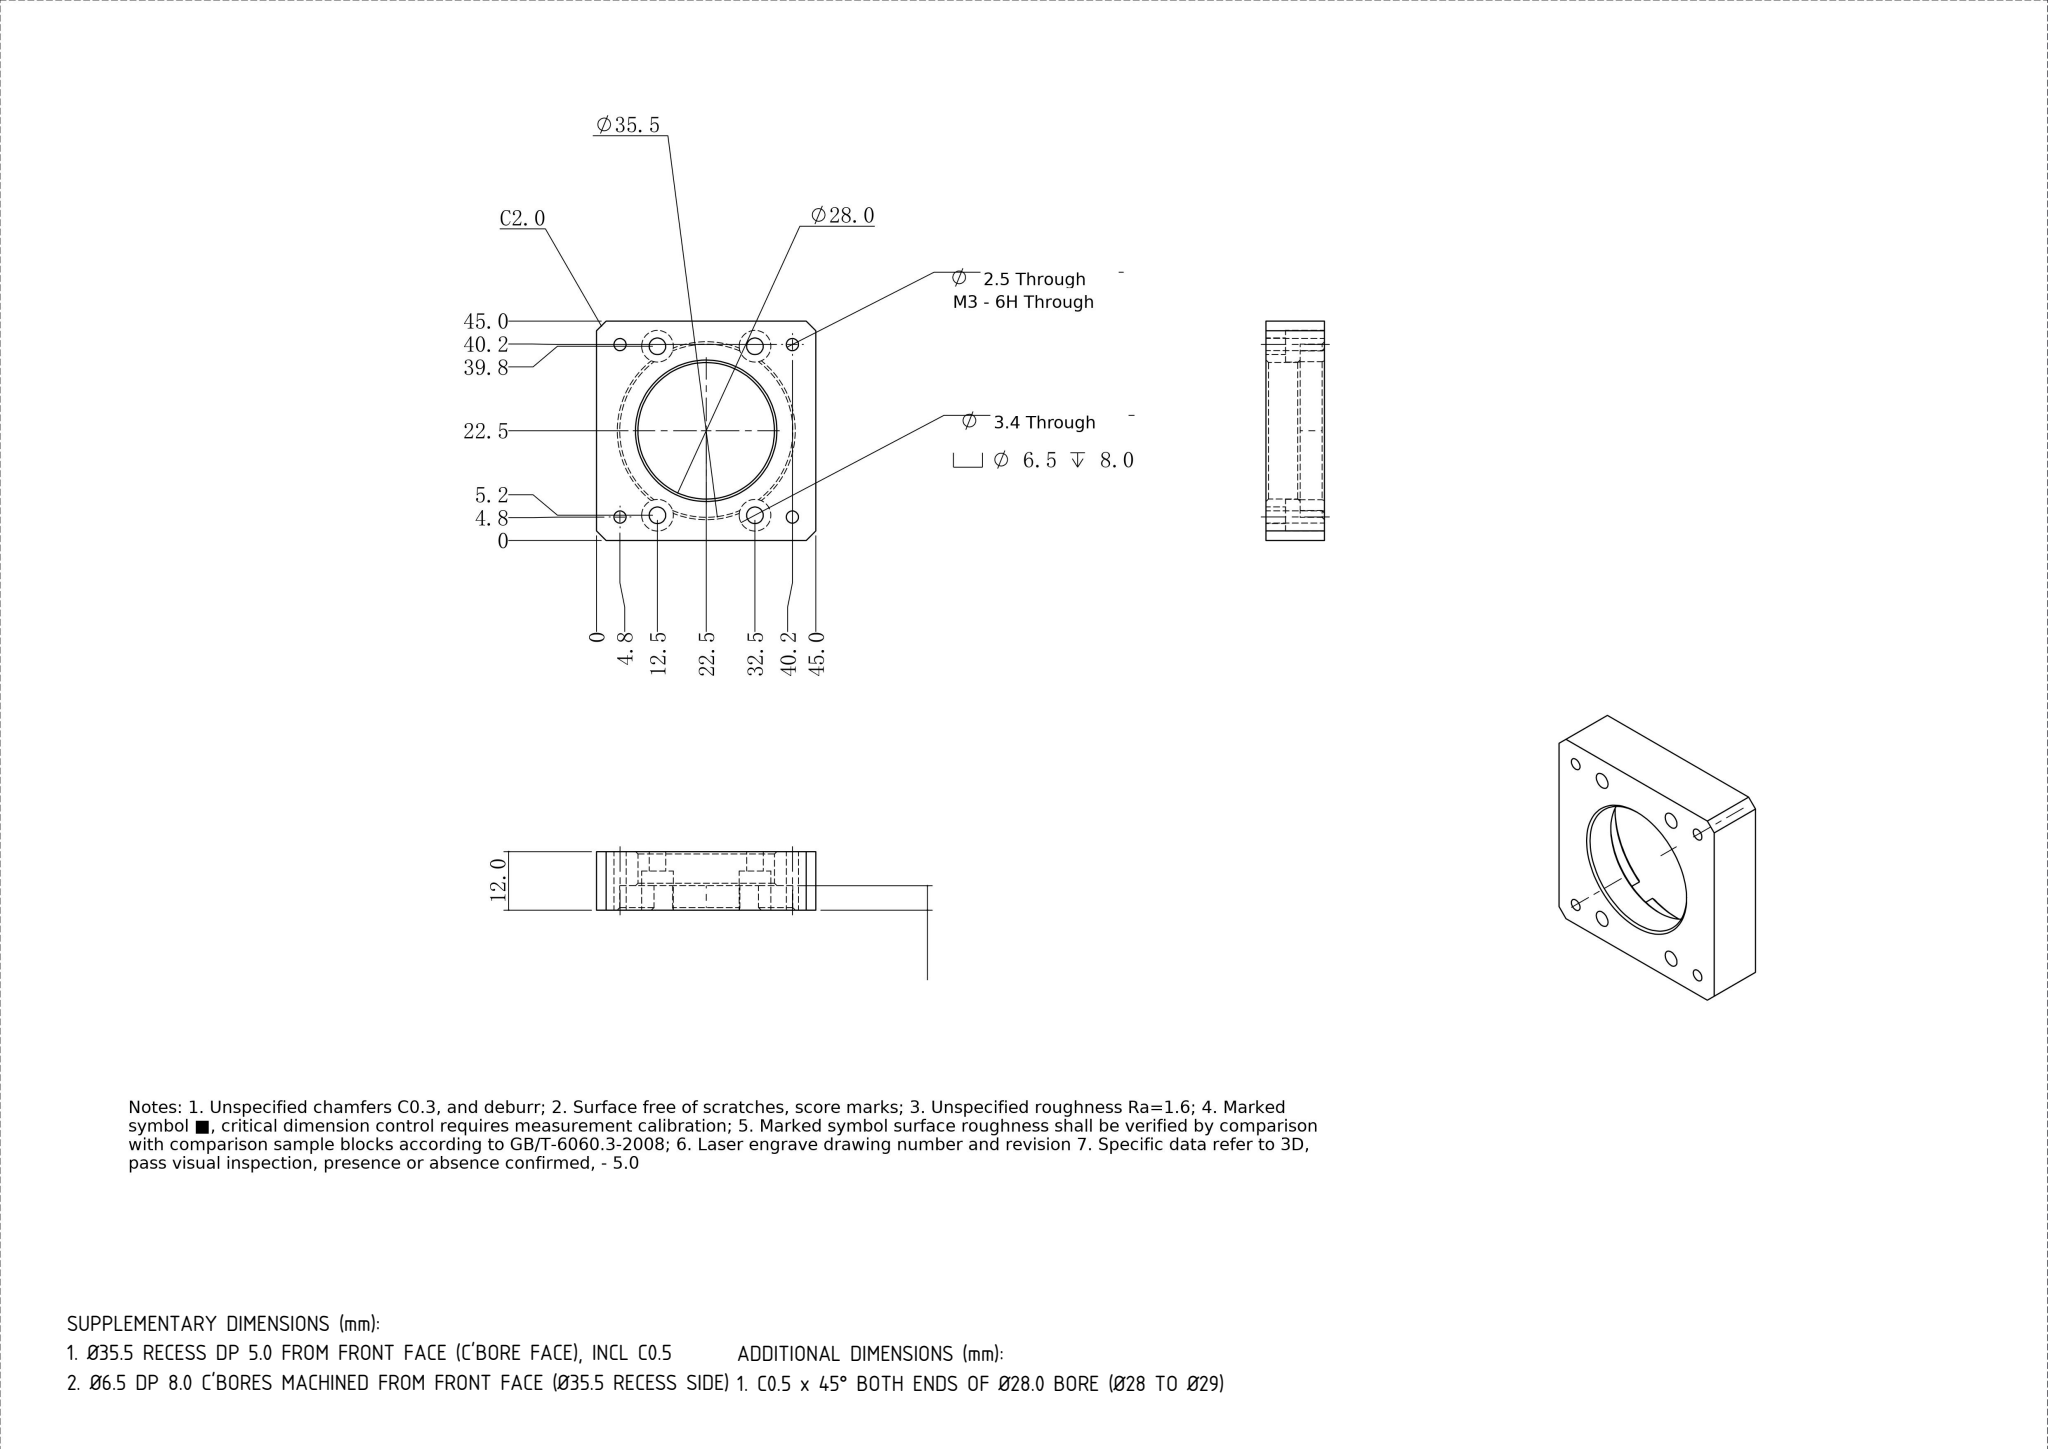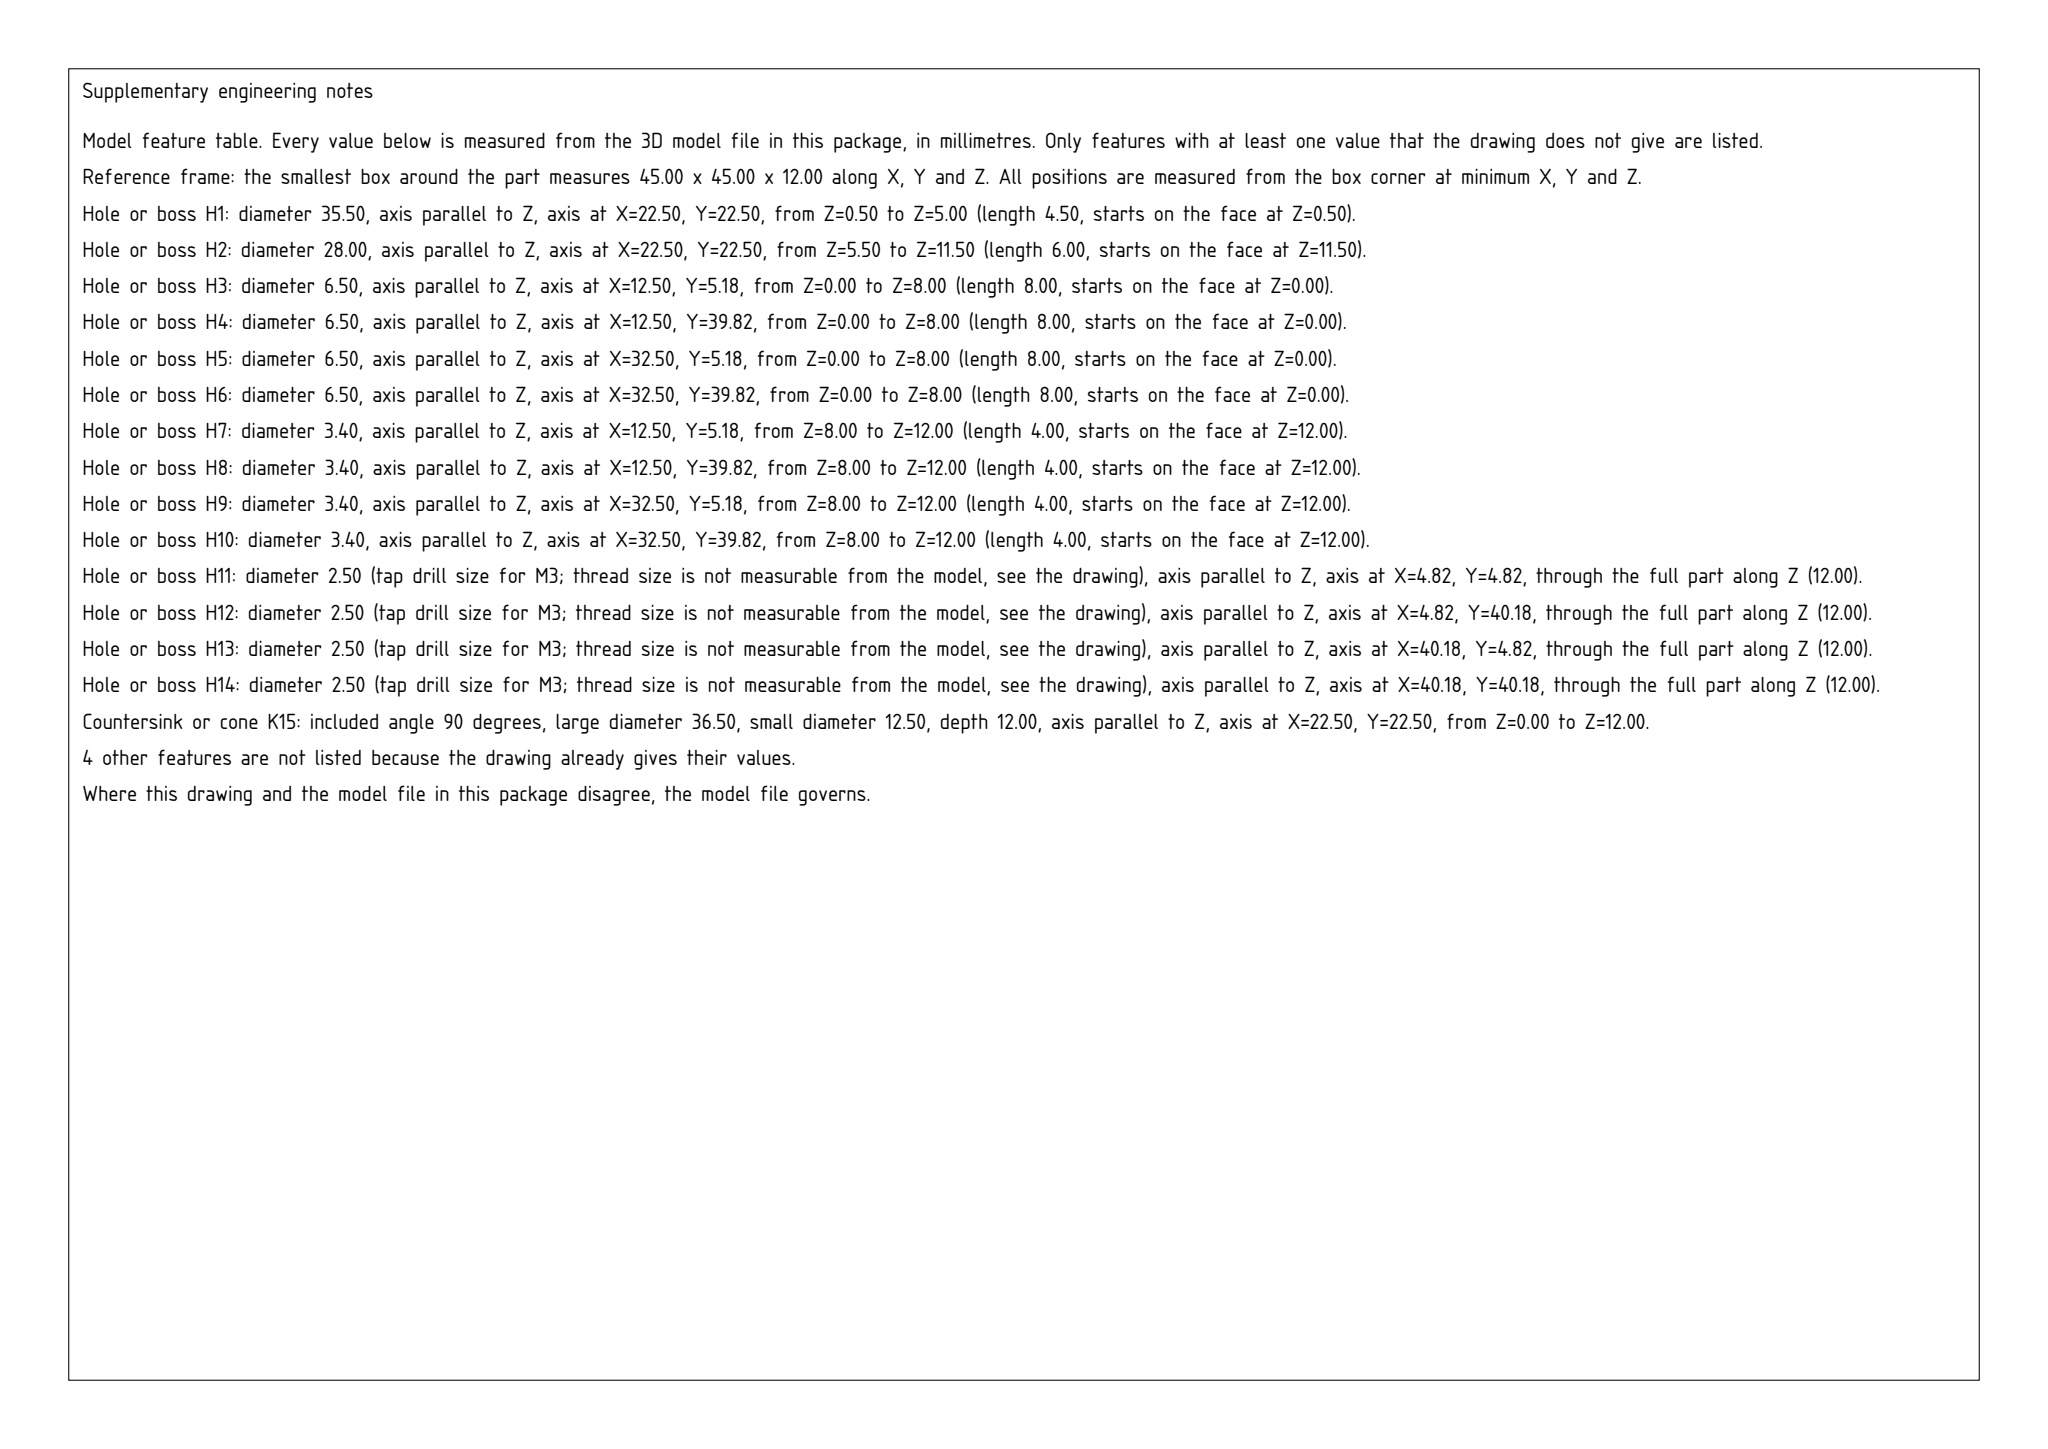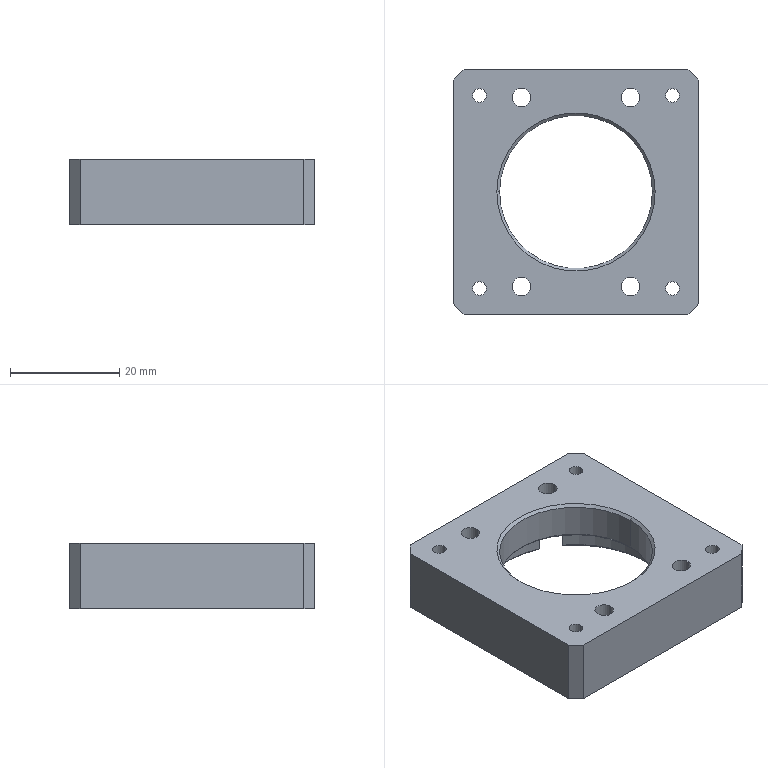Part | SolidWorks | mm | 1 solid | 55 faces | box 45 x 45 x 12 mm | volume 13528 mm3 | cylinder 31 | plane 15 | cone 9 | commonest cylinder face diameters 3.4 x8 6.5 x8 2.5 x8 35.5 x5 28 x2
build123d program:
from build123d import *

# Parameters (mm, degrees)
SKETCH1_W                                       = 45
SKETCH1_H                                       = 45
BOSS_EXTRUDE1_DEPTH                             = 6
SKETCH2_R                                       = 17.75
CUT_EXTRUDE1_DEPTH                              = 5
SKETCH7_R                                       = 14
CUT_EXTRUDE2_DEPTH                              = 33.581
M3_TAPPED_HOLE1_D                               = 2.5
M3_HEX_SOCKET_HEAD_CAP_SCREW_CBORE1_D           = 3.4
M3_HEX_SOCKET_HEAD_CAP_SCREW_CBORE1_CBORE_D     = 6.5
M3_HEX_SOCKET_HEAD_CAP_SCREW_CBORE1_CBORE_DEPTH = 8
CHAMFER1_SIZE                                   = 2
CHAMFER2_SIZE                                   = 0.5


with BuildPart() as part:
    # Sketch1 → Boss-Extrude1 (new, symmetric)
    with BuildSketch(Plane.XY):
        Rectangle(SKETCH1_W, SKETCH1_H)
    extrude(amount=BOSS_EXTRUDE1_DEPTH, both=True)

    # Sketch2 → Cut-Extrude1 (cut)
    with BuildSketch(Plane(origin=(0, 0, -6), x_dir=(-1, 0, 0), z_dir=(0, 0, -1))):
        Circle(SKETCH2_R)
    extrude(amount=-CUT_EXTRUDE1_DEPTH, mode=Mode.SUBTRACT)

    # Sketch7 → Cut-Extrude2 (cut, through all)
    with BuildSketch(Plane(origin=(0, 0, -1), x_dir=(-1, 0, 0), z_dir=(0, 0, -1))):
        Circle(SKETCH7_R)
    extrude(amount=-CUT_EXTRUDE2_DEPTH, mode=Mode.SUBTRACT)

    # M3 Tapped Hole1 (through all)
    with Locations(Plane(origin=(0, 0, -6), x_dir=(-1, 0, 0), z_dir=(0, 0, -1))):
        with Locations((17.678, -17.678), (-17.678, 17.678), (-17.678, -17.678), (17.678, 17.678)):
            Hole(M3_TAPPED_HOLE1_D / 2)

    # M3 Hex Socket Head Cap Screw CBORE1 (through all)
    with Locations(Plane(origin=(0, 0, -6), x_dir=(-1, 0, 0), z_dir=(0, 0, -1))):
        with Locations((10, -17.321), (-10, -17.321), (10, 17.321), (-10, 17.321)):
            CounterBoreHole(M3_HEX_SOCKET_HEAD_CAP_SCREW_CBORE1_D / 2, M3_HEX_SOCKET_HEAD_CAP_SCREW_CBORE1_CBORE_D / 2, M3_HEX_SOCKET_HEAD_CAP_SCREW_CBORE1_CBORE_DEPTH)

    # Chamfer1
    chamfer1_edges = [part.edges().sort_by_distance(p)[0] for p in [
        (22.5, -22.5, 0),
        (-22.5, -22.5, 0),
        (-22.5, 22.5, 0),
        (22.5, 22.5, 0),
    ]]
    chamfer(chamfer1_edges, length=CHAMFER1_SIZE)

    # Chamfer2
    chamfer2_edges = [part.edges().sort_by_distance(p)[0] for p in [
        (14, 0, 6),
        (14, 0, -1),
        (17.75, 0, -6),
        (0, 17.75, -6),
        (0, -17.75, -6),
        (-17.75, 0, -6),
    ]]
    chamfer(chamfer2_edges, length=CHAMFER2_SIZE)


solid = part.part